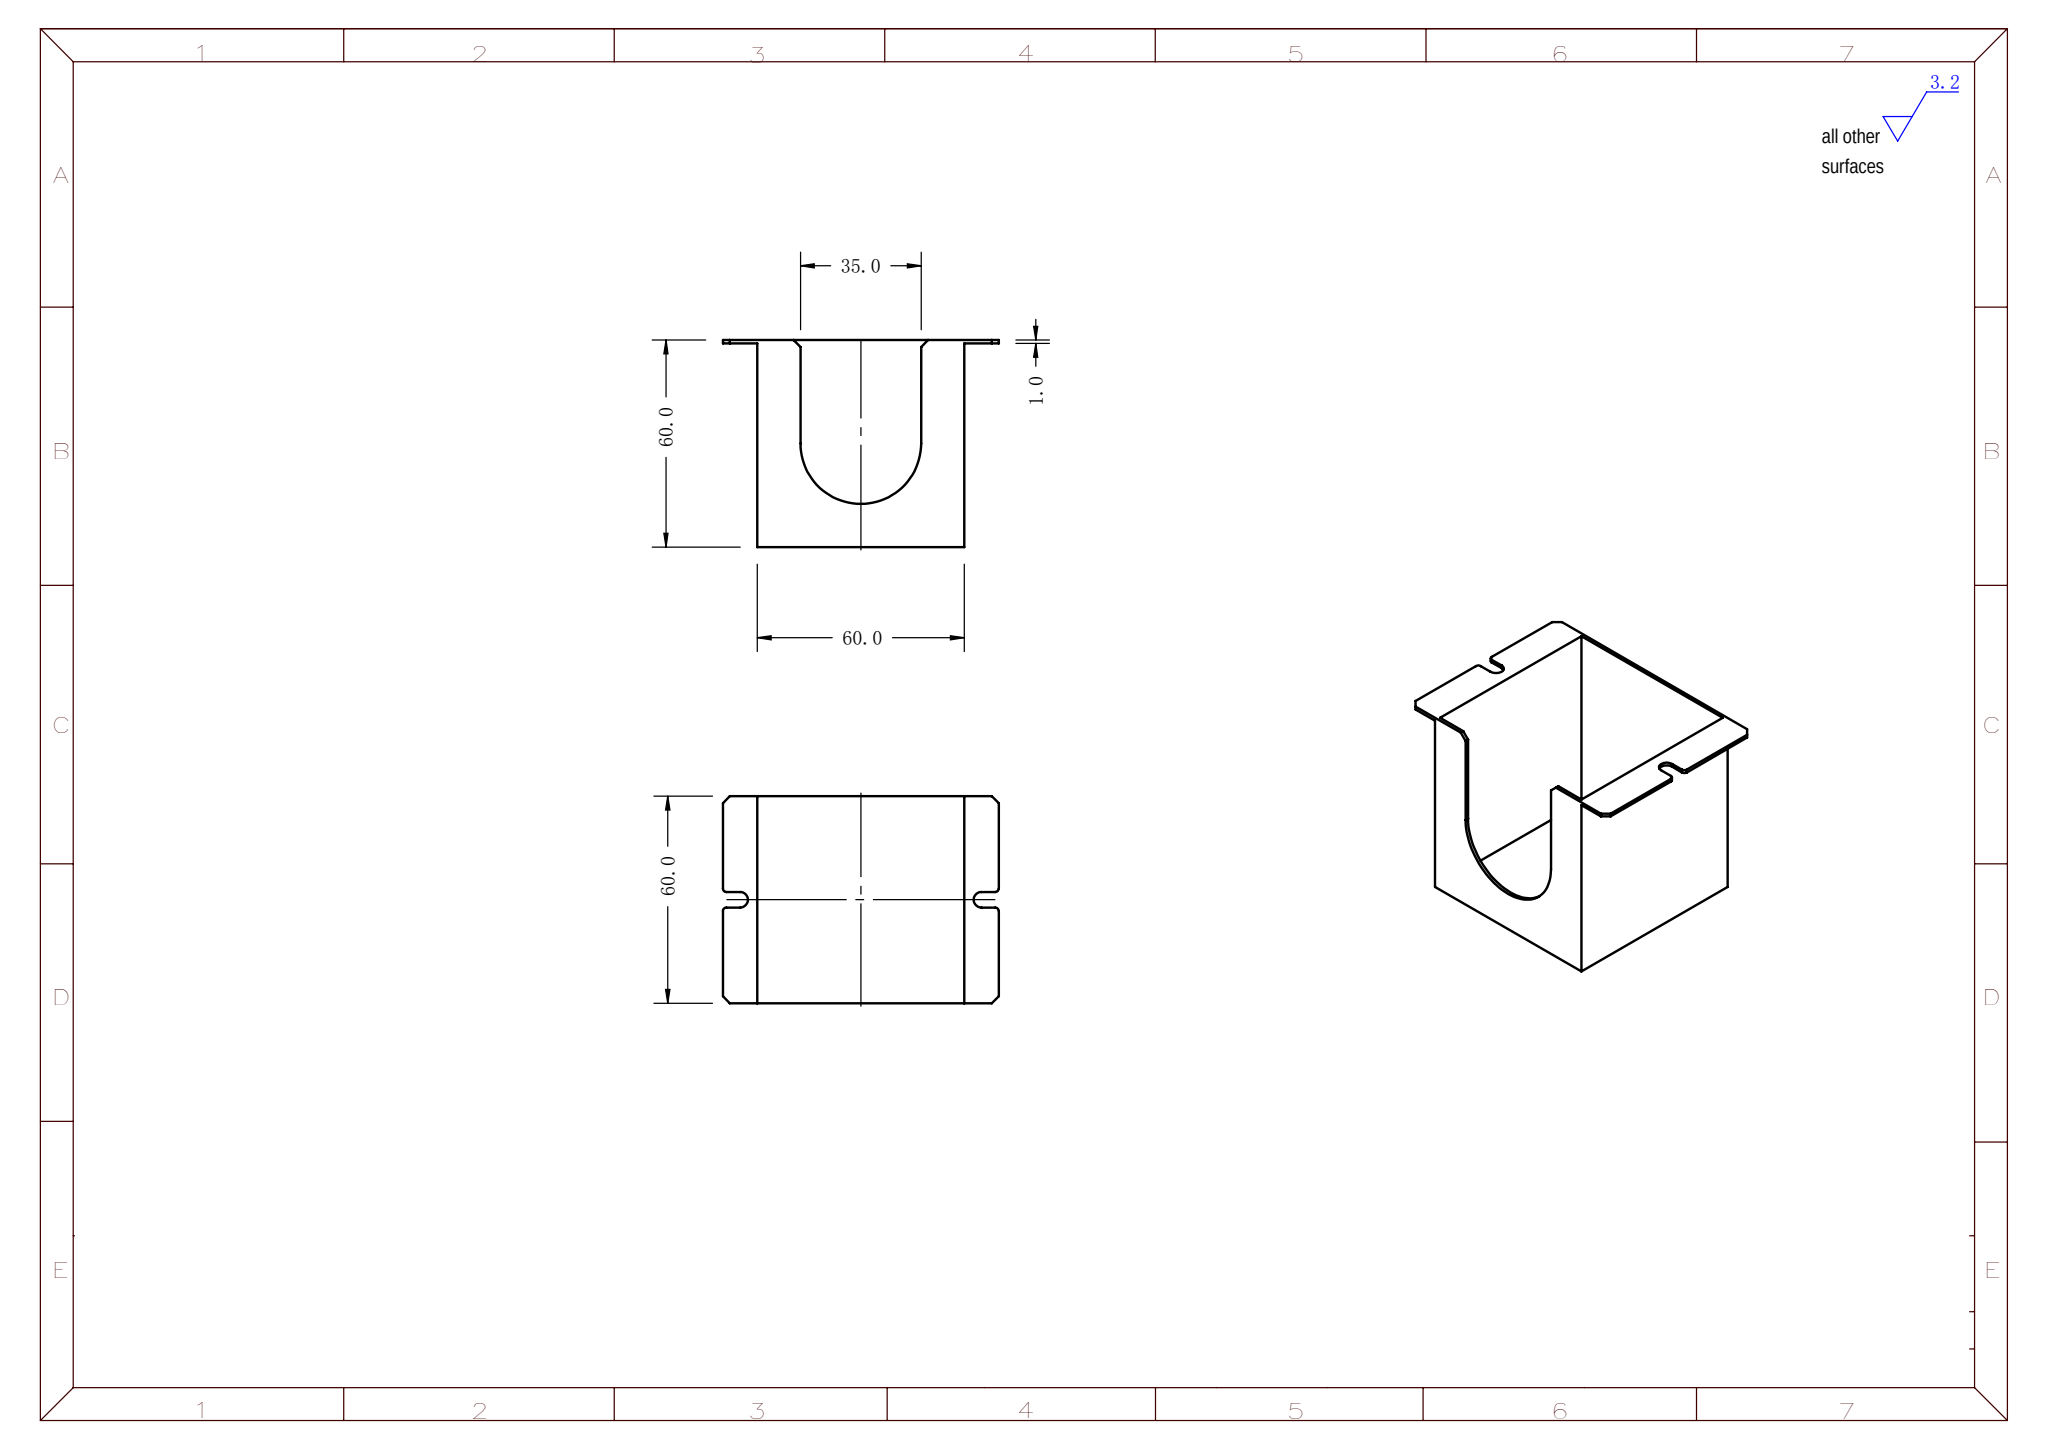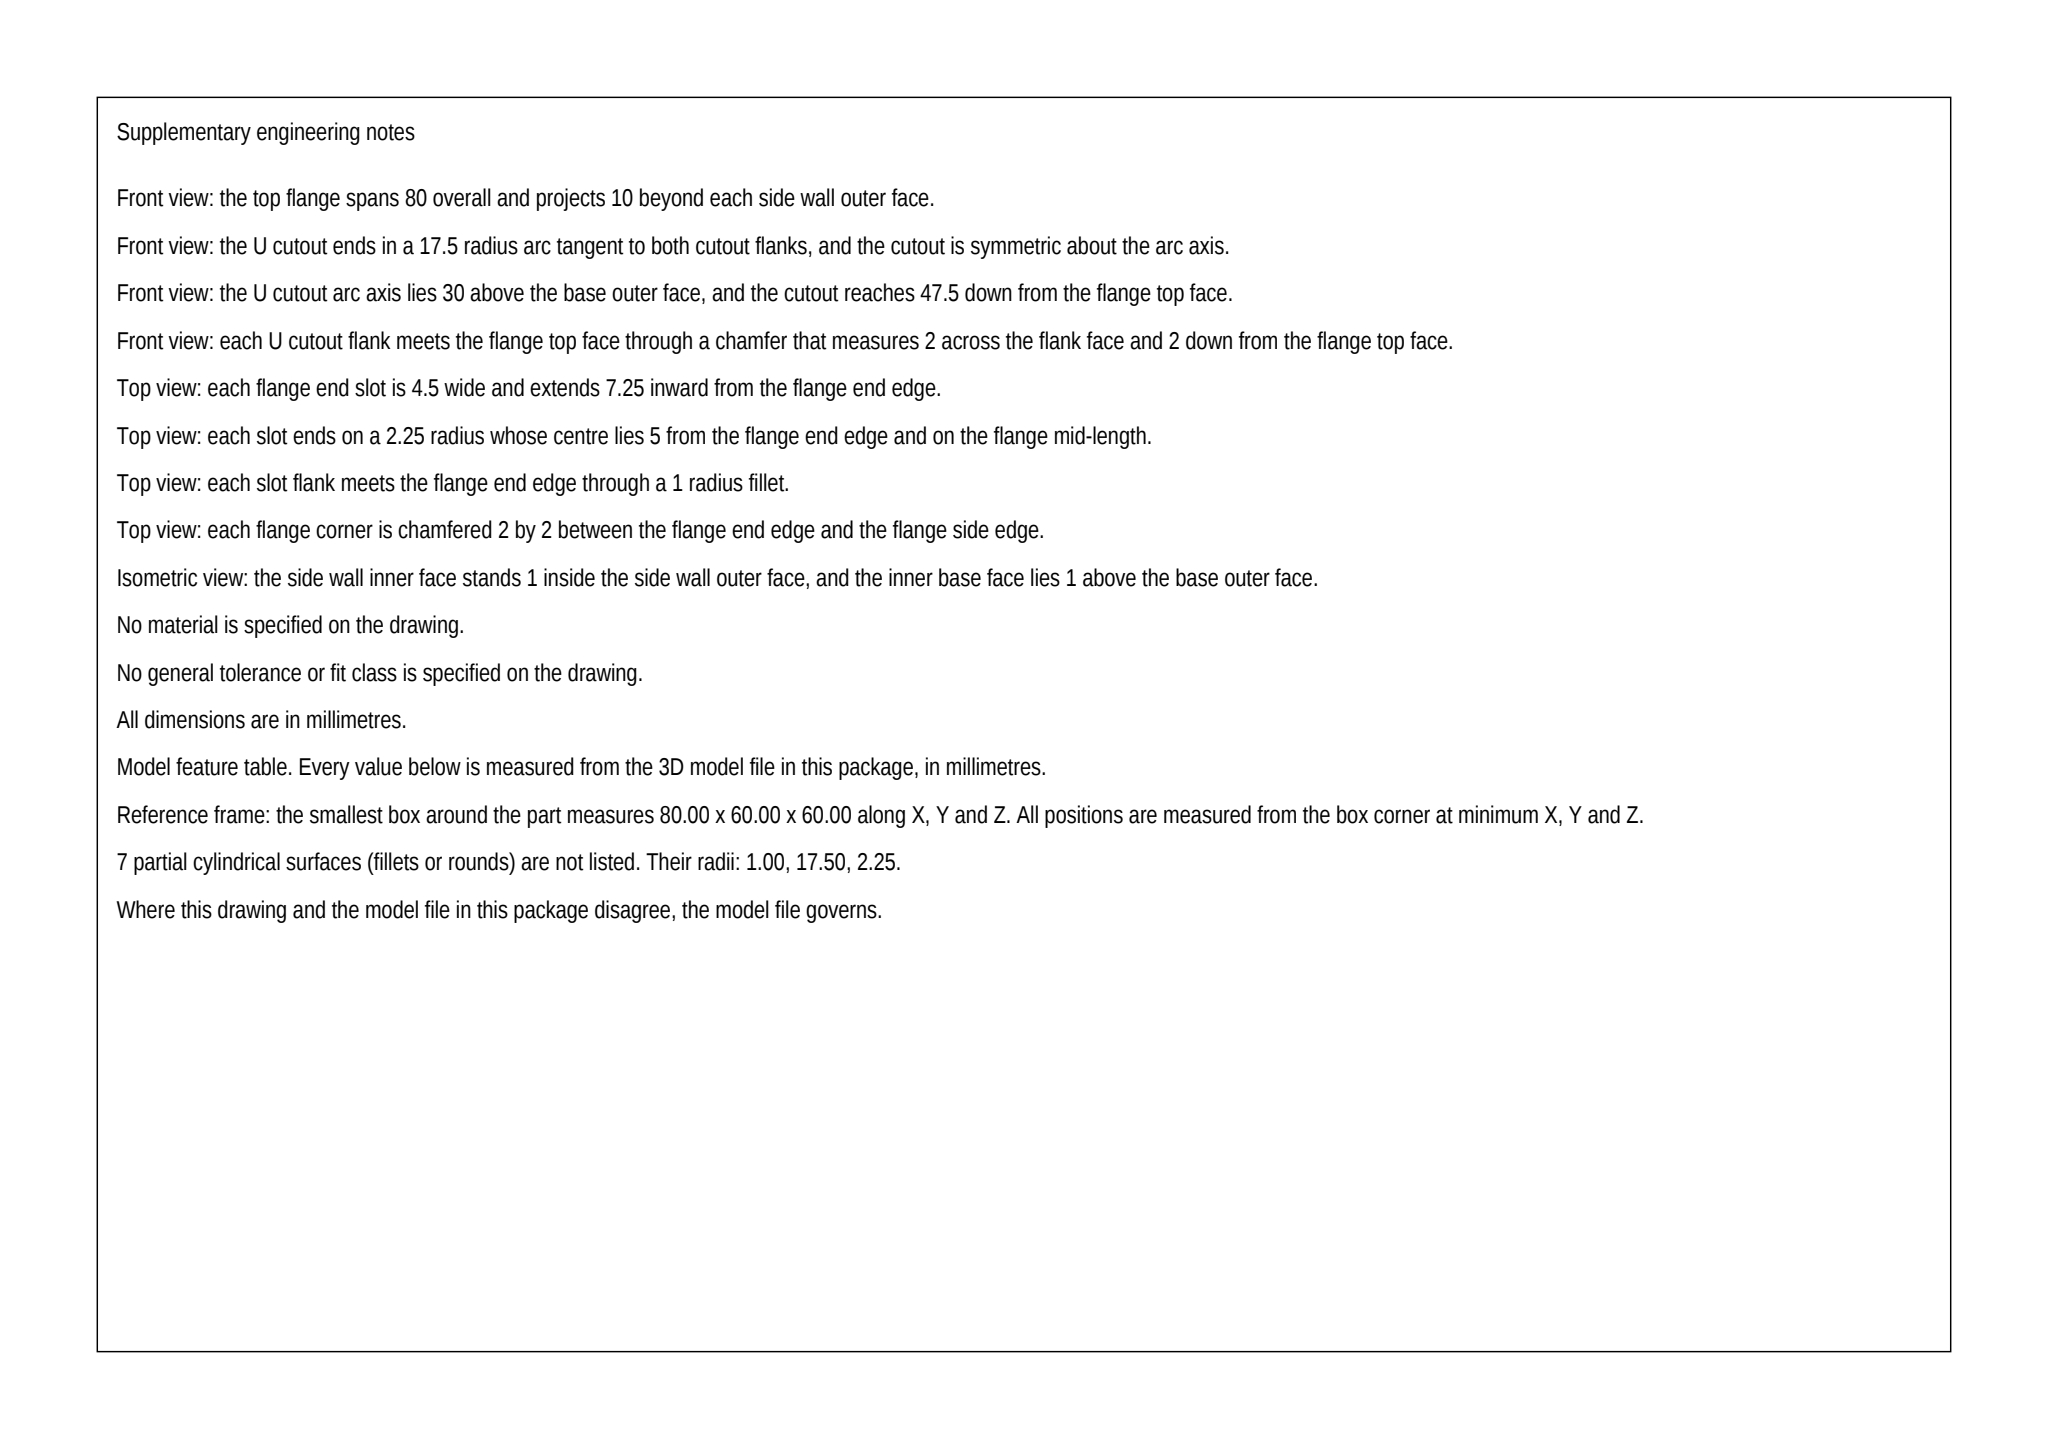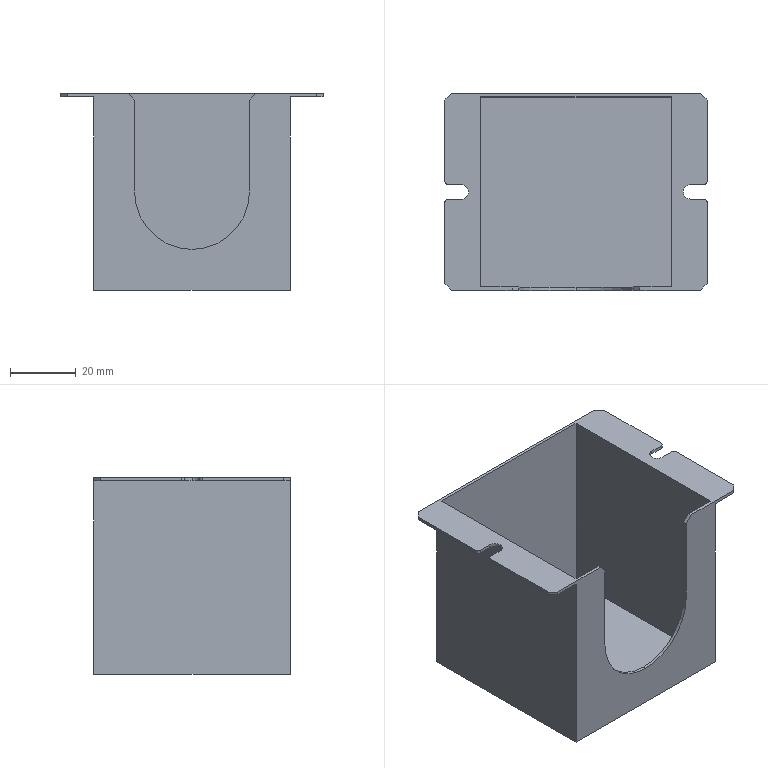Part | SolidWorks | mm | 1 solid | 38 faces | box 80 x 60 x 60 mm | volume 17119 mm3 | plane 29 | cylinder 9 | commonest cylinder face diameters 2 x4 4.5 x3 35 x2
Drawing notes:
OVERALL LG 80 ACROSS FLANGES; FLANGE PROJ 10 EA SIDE OF 60 BODY | from the solid: bbox_xyz x=80; wall planes x=10 & x=70 give 60 body, 10 flange each side
U-SLOT 35 WIDE, ARC C/L 30 UP FROM BTM, SLOT BTM 12.5 UP FROM BTM | from the solid: cyl dia 35 axis y at [x40,z30]; 30-17.5=12.5 above z=0
FLANGE NOTCH 4.5 WIDE, CTRD ON 60 WIDTH (y=27.75/32.25) | from the solid: cyl dia 4.5 at y=30; planes y=27.75 & y=32.25
NOTCH END FULL R2.25; 4X Ø2.0 RELIEF HOLES TANG TO NOTCH SIDES | from the solid: dia 4.5 cyl (R2.25) at x=5/75; dia 2.0 cyl at x=1/79, y=26.75/33.25
NOTCH C/L 30 FROM EA SIDE; Ø2.0 RELIEF HOLE C/L 1 FROM FLANGE EDGE | from the solid: dia4.5 cyl pos [5,30] & [75,30]; dia2.0 holes at x=1 and x=79
NOTCH DEPTH 7.25 FROM FLANGE EDGE, END R2.25 C/L 5 FROM EDGE | from the solid: dia 4.5 cyl axis at x=5 (and x=75); 5+2.25=7.25 from x=0 / x=80
2X Ø35 U-SLOT: IN BOTH FRONT & REAR 1.0 WALLS, ON CL | from the solid: cylinders [35.0,'y',[40.0,null,30.0],1.0,count 2]; walls y=0-1 and y=59-60